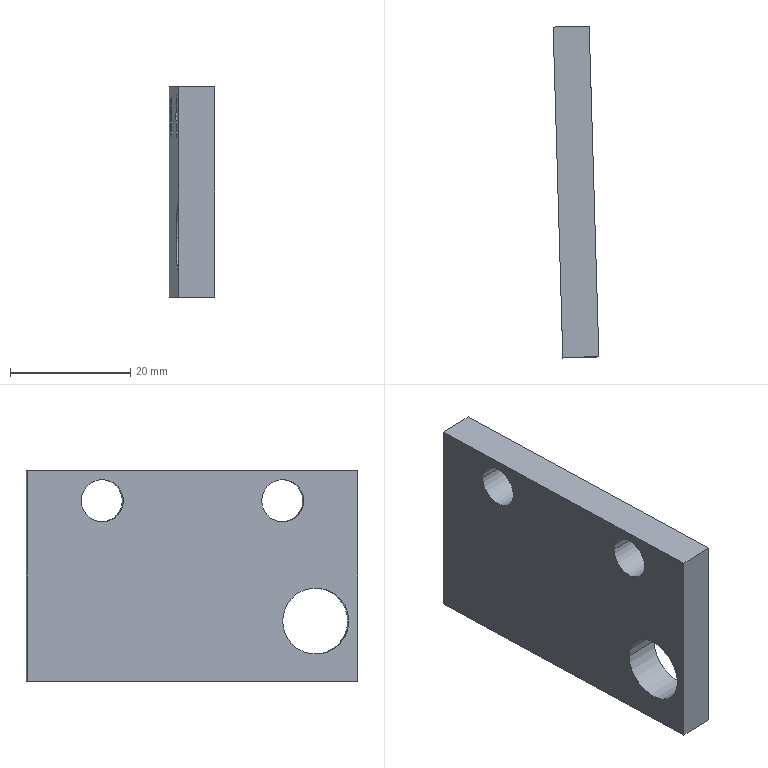Component | SolidWorks | BufferPad-2 | 1 solid | 12 faces | box 7.6 x 55.15 x 35 mm | volume 10518 mm3 | cylinder 6 | plane 6 | commonest cylinder face diameters 7 x4 11 x2 | material 6063
build123d program:
from build123d import *

# Parameters (mm, degrees)
SKETCH1_W           = 55
SKETCH1_H           = 35
BOSS_EXTRUDE1_DEPTH = 6
SKETCH2_R           = 3.5
CUT_EXTRUDE1_DEPTH  = 34.144
SKETCH3_R           = 5.5
CUT_EXTRUDE2_DEPTH  = 34.144


with BuildPart() as part:
    # Sketch1 → Boss-Extrude1 (new body)
    with BuildSketch(Plane.XY):
        Rectangle(SKETCH1_W, SKETCH1_H)
    extrude(amount=BOSS_EXTRUDE1_DEPTH)

    # Sketch2 → Cut-Extrude1 (cut, through all)
    with BuildSketch(Plane.XY.offset(6)):
        with Locations((-15, -12.5)):
            Circle(SKETCH2_R)
        with Locations((15, -12.5)):
            Circle(SKETCH2_R)
    extrude(amount=-CUT_EXTRUDE1_DEPTH, mode=Mode.SUBTRACT)

    # Sketch3 → Cut-Extrude2 (cut, through all)
    with BuildSketch(Plane.XY.offset(6)):
        with Locations((-20.5, 7.5)):
            Circle(SKETCH3_R)
    extrude(amount=-CUT_EXTRUDE2_DEPTH, mode=Mode.SUBTRACT)


solid = part.part

# Placed as in the assembly
solid = solid.moved(Location((-13.559, -152.418, -1233.71), (90, -88.328, 180)))
STEP:
#1=CARTESIAN_POINT('',(-0.504,-7.024,-48.867));
#2=VERTEX_POINT('',#1);
#3=CARTESIAN_POINT('',(-0.5166,-6.591,-48.867));
#4=VERTEX_POINT('',#3);
#5=CARTESIAN_POINT('',(-0.5103,-6.807,-48.867));
#6=DIRECTION('',(-0.9996,-0.02918,0.));
#7=DIRECTION('',(-0.02918,0.9996,0.));
#8=AXIS2_PLACEMENT_3D('',#5,#6,#7);
#9=CIRCLE('',#8,0.2165);
#10=EDGE_CURVE('',#2,#4,#9,.T.);
#11=ORIENTED_EDGE('',*,*,#10,.F.);
#12=CARTESIAN_POINT('',(-0.7401,-7.031,-48.867));
#13=VERTEX_POINT('',#12);
#14=CARTESIAN_POINT('',(-0.504,-7.024,-48.867));
#15=DIRECTION('',(-0.9996,-0.02918,0.));
#16=VECTOR('',#15,39.37);
#17=LINE('',#14,#16);
#18=EDGE_CURVE('',#2,#13,#17,.T.);
#19=ORIENTED_EDGE('',*,*,#18,.T.);
#20=CARTESIAN_POINT('',(-0.7527,-6.598,-48.867));
#21=VERTEX_POINT('',#20);
#22=CARTESIAN_POINT('',(-0.7464,-6.814,-48.867));
#23=DIRECTION('',(-0.9996,-0.02918,0.));
#24=DIRECTION('',(-0.02918,0.9996,0.));
#25=AXIS2_PLACEMENT_3D('',#22,#23,#24);
#26=CIRCLE('',#25,0.2165);
#27=EDGE_CURVE('',#13,#21,#26,.T.);
#28=ORIENTED_EDGE('',*,*,#27,.T.);
#29=CARTESIAN_POINT('',(-0.5166,-6.591,-48.867));
#30=DIRECTION('',(-0.9996,-0.02918,0.));
#31=VECTOR('',#30,39.37);
#32=LINE('',#29,#31);
#33=EDGE_CURVE('',#4,#21,#32,.T.);
#34=ORIENTED_EDGE('',*,*,#33,.F.);
#35=EDGE_LOOP('',(#11,#19,#28,#34));
#36=FACE_OUTER_BOUND('',#35,.T.);
#37=CARTESIAN_POINT('',(-0.5103,-6.807,-48.867));
#38=DIRECTION('',(-0.9996,-0.02918,0.));
#39=DIRECTION('',(-0.02918,0.9996,0.));
#40=AXIS2_PLACEMENT_3D('',#37,#38,#39);
#41=CYLINDRICAL_SURFACE('',#40,0.2165);
#42=ADVANCED_FACE('',(#36),#41,.F.);
#43=CARTESIAN_POINT('',(-0.547,-5.548,-48.079));
#44=VERTEX_POINT('',#43);
#45=CARTESIAN_POINT('',(-0.5551,-5.273,-48.079));
#46=VERTEX_POINT('',#45);
#47=CARTESIAN_POINT('',(-0.5511,-5.41,-48.079));
#48=DIRECTION('',(-0.9996,-0.02918,0.));
#49=DIRECTION('',(-0.02918,0.9996,0.));
#50=AXIS2_PLACEMENT_3D('',#47,#48,#49);
#51=CIRCLE('',#50,0.1378);
#52=EDGE_CURVE('',#44,#46,#51,.T.);
#53=ORIENTED_EDGE('',*,*,#52,.F.);
#54=CARTESIAN_POINT('',(-0.7832,-5.555,-48.079));
#55=VERTEX_POINT('',#54);
#56=CARTESIAN_POINT('',(-0.547,-5.548,-48.079));
#57=DIRECTION('',(-0.9996,-0.02918,0.));
#58=VECTOR('',#57,39.37);
#59=LINE('',#56,#58);
#60=EDGE_CURVE('',#44,#55,#59,.T.);
#61=ORIENTED_EDGE('',*,*,#60,.T.);
#62=CARTESIAN_POINT('',(-0.7912,-5.28,-48.079));
#63=VERTEX_POINT('',#62);
#64=CARTESIAN_POINT('',(-0.7872,-5.417,-48.079));
#65=DIRECTION('',(-0.9996,-0.02918,0.));
#66=DIRECTION('',(-0.02918,0.9996,0.));
#67=AXIS2_PLACEMENT_3D('',#64,#65,#66);
#68=CIRCLE('',#67,0.1378);
#69=EDGE_CURVE('',#55,#63,#68,.T.);
#70=ORIENTED_EDGE('',*,*,#69,.T.);
#71=CARTESIAN_POINT('',(-0.5551,-5.273,-48.079));
#72=DIRECTION('',(-0.9996,-0.02918,0.));
#73=VECTOR('',#72,39.37);
#74=LINE('',#71,#73);
#75=EDGE_CURVE('',#46,#63,#74,.T.);
#76=ORIENTED_EDGE('',*,*,#75,.F.);
#77=EDGE_LOOP('',(#53,#61,#70,#76));
#78=FACE_OUTER_BOUND('',#77,.T.);
#79=CARTESIAN_POINT('',(-0.5511,-5.41,-48.079));
#80=DIRECTION('',(-0.9996,-0.02918,0.));
#81=DIRECTION('',(-0.02918,0.9996,0.));
#82=AXIS2_PLACEMENT_3D('',#79,#80,#81);
#83=CYLINDRICAL_SURFACE('',#82,0.1378);
#84=ADVANCED_FACE('',(#78),#83,.F.);
#85=CARTESIAN_POINT('',(-0.5126,-6.729,-48.079));
#86=VERTEX_POINT('',#85);
#87=CARTESIAN_POINT('',(-0.5206,-6.453,-48.079));
#88=VERTEX_POINT('',#87);
#89=CARTESIAN_POINT('',(-0.5166,-6.591,-48.079));
#90=DIRECTION('',(-0.9996,-0.02918,0.));
#91=DIRECTION('',(-0.02918,0.9996,0.));
#92=AXIS2_PLACEMENT_3D('',#89,#90,#91);
#93=CIRCLE('',#92,0.1378);
#94=EDGE_CURVE('',#86,#88,#93,.T.);
#95=ORIENTED_EDGE('',*,*,#94,.F.);
#96=CARTESIAN_POINT('',(-0.7487,-6.736,-48.079));
#97=VERTEX_POINT('',#96);
#98=CARTESIAN_POINT('',(-0.5126,-6.729,-48.079));
#99=DIRECTION('',(-0.9996,-0.02918,0.));
#100=VECTOR('',#99,39.37);
#101=LINE('',#98,#100);
#102=EDGE_CURVE('',#86,#97,#101,.T.);
#103=ORIENTED_EDGE('',*,*,#102,.T.);
#104=CARTESIAN_POINT('',(-0.7567,-6.46,-48.079));
#105=VERTEX_POINT('',#104);
#106=CARTESIAN_POINT('',(-0.7527,-6.598,-48.079));
#107=DIRECTION('',(-0.9996,-0.02918,0.));
#108=DIRECTION('',(-0.02918,0.9996,0.));
#109=AXIS2_PLACEMENT_3D('',#106,#107,#108);
#110=CIRCLE('',#109,0.1378);
#111=EDGE_CURVE('',#97,#105,#110,.T.);
#112=ORIENTED_EDGE('',*,*,#111,.T.);
#113=CARTESIAN_POINT('',(-0.5206,-6.453,-48.079));
#114=DIRECTION('',(-0.9996,-0.02918,0.));
#115=VECTOR('',#114,39.37);
#116=LINE('',#113,#115);
#117=EDGE_CURVE('',#88,#105,#116,.T.);
#118=ORIENTED_EDGE('',*,*,#117,.F.);
#119=EDGE_LOOP('',(#95,#103,#112,#118));
#120=FACE_OUTER_BOUND('',#119,.T.);
#121=CARTESIAN_POINT('',(-0.5166,-6.591,-48.079));
#122=DIRECTION('',(-0.9996,-0.02918,0.));
#123=DIRECTION('',(-0.02918,0.9996,0.));
#124=AXIS2_PLACEMENT_3D('',#121,#122,#123);
#125=CYLINDRICAL_SURFACE('',#124,0.1378);
#126=ADVANCED_FACE('',(#120),#125,.F.);
#127=CARTESIAN_POINT('',(-0.5654,-4.919,-47.882));
#128=VERTEX_POINT('',#127);
#129=CARTESIAN_POINT('',(-0.5654,-4.919,-49.26));
#130=VERTEX_POINT('',#129);
#131=CARTESIAN_POINT('',(-0.5654,-4.919,-49.26));
#132=DIRECTION('',(-0.,0.,-1.));
#133=VECTOR('',#132,39.37);
#134=LINE('',#131,#133);
#135=EDGE_CURVE('',#128,#130,#134,.T.);
#136=ORIENTED_EDGE('',*,*,#135,.T.);
#137=CARTESIAN_POINT('',(-0.8015,-4.925,-49.26));
#138=VERTEX_POINT('',#137);
#139=CARTESIAN_POINT('',(-0.8015,-4.925,-49.26));
#140=DIRECTION('',(0.9996,0.02918,-0.));
#141=VECTOR('',#140,39.37);
#142=LINE('',#139,#141);
#143=EDGE_CURVE('',#138,#130,#142,.T.);
#144=ORIENTED_EDGE('',*,*,#143,.F.);
#145=CARTESIAN_POINT('',(-0.8015,-4.925,-47.882));
#146=VERTEX_POINT('',#145);
#147=CARTESIAN_POINT('',(-0.8015,-4.925,-49.26));
#148=DIRECTION('',(-0.,0.,-1.));
#149=VECTOR('',#148,39.37);
#150=LINE('',#147,#149);
#151=EDGE_CURVE('',#146,#138,#150,.T.);
#152=ORIENTED_EDGE('',*,*,#151,.F.);
#153=CARTESIAN_POINT('',(-0.8015,-4.925,-47.882));
#154=DIRECTION('',(0.9996,0.02918,-0.));
#155=VECTOR('',#154,39.37);
#156=LINE('',#153,#155);
#157=EDGE_CURVE('',#146,#128,#156,.T.);
#158=ORIENTED_EDGE('',*,*,#157,.T.);
#159=EDGE_LOOP('',(#136,#144,#152,#158));
#160=FACE_OUTER_BOUND('',#159,.T.);
#161=CARTESIAN_POINT('',(-0.8015,-4.925,-49.26));
#162=DIRECTION('',(0.02918,-0.9996,-0.));
#163=DIRECTION('',(0.,-0.,1.));
#164=AXIS2_PLACEMENT_3D('',#161,#162,#163);
#165=PLANE('',#164);
#166=ADVANCED_FACE('',(#160),#165,.F.);
#167=CARTESIAN_POINT('',(-0.5022,-7.083,-49.26));
#168=VERTEX_POINT('',#167);
#169=CARTESIAN_POINT('',(-0.5022,-7.083,-49.26));
#170=DIRECTION('',(0.02918,-0.9996,-0.));
#171=VECTOR('',#170,39.37);
#172=LINE('',#169,#171);
#173=EDGE_CURVE('',#130,#168,#172,.T.);
#174=ORIENTED_EDGE('',*,*,#173,.T.);
#175=CARTESIAN_POINT('',(-0.7384,-7.09,-49.26));
#176=VERTEX_POINT('',#175);
#177=CARTESIAN_POINT('',(-0.7384,-7.09,-49.26));
#178=DIRECTION('',(0.9996,0.02918,-0.));
#179=VECTOR('',#178,39.37);
#180=LINE('',#177,#179);
#181=EDGE_CURVE('',#176,#168,#180,.T.);
#182=ORIENTED_EDGE('',*,*,#181,.F.);
#183=CARTESIAN_POINT('',(-0.7384,-7.09,-49.26));
#184=DIRECTION('',(0.02918,-0.9996,-0.));
#185=VECTOR('',#184,39.37);
#186=LINE('',#183,#185);
#187=EDGE_CURVE('',#138,#176,#186,.T.);
#188=ORIENTED_EDGE('',*,*,#187,.F.);
#189=ORIENTED_EDGE('',*,*,#143,.T.);
#190=EDGE_LOOP('',(#174,#182,#188,#189));
#191=FACE_OUTER_BOUND('',#190,.T.);
#192=CARTESIAN_POINT('',(-0.7384,-7.09,-49.26));
#193=DIRECTION('',(0.,-0.,1.));
#194=DIRECTION('',(0.9996,0.02918,-0.));
#195=AXIS2_PLACEMENT_3D('',#192,#193,#194);
#196=PLANE('',#195);
#197=ADVANCED_FACE('',(#191),#196,.F.);
#198=CARTESIAN_POINT('',(-0.5022,-7.083,-47.882));
#199=VERTEX_POINT('',#198);
#200=CARTESIAN_POINT('',(-0.5022,-7.083,-49.26));
#201=DIRECTION('',(0.,-0.,1.));
#202=VECTOR('',#201,39.37);
#203=LINE('',#200,#202);
#204=EDGE_CURVE('',#168,#199,#203,.T.);
#205=ORIENTED_EDGE('',*,*,#204,.T.);
#206=CARTESIAN_POINT('',(-0.7384,-7.09,-47.882));
#207=VERTEX_POINT('',#206);
#208=CARTESIAN_POINT('',(-0.7384,-7.09,-47.882));
#209=DIRECTION('',(0.9996,0.02918,-0.));
#210=VECTOR('',#209,39.37);
#211=LINE('',#208,#210);
#212=EDGE_CURVE('',#207,#199,#211,.T.);
#213=ORIENTED_EDGE('',*,*,#212,.F.);
#214=CARTESIAN_POINT('',(-0.7384,-7.09,-49.26));
#215=DIRECTION('',(0.,-0.,1.));
#216=VECTOR('',#215,39.37);
#217=LINE('',#214,#216);
#218=EDGE_CURVE('',#176,#207,#217,.T.);
#219=ORIENTED_EDGE('',*,*,#218,.F.);
#220=ORIENTED_EDGE('',*,*,#181,.T.);
#221=EDGE_LOOP('',(#205,#213,#219,#220));
#222=FACE_OUTER_BOUND('',#221,.T.);
#223=CARTESIAN_POINT('',(-0.7384,-7.09,-49.26));
#224=DIRECTION('',(-0.02918,0.9996,0.));
#225=DIRECTION('',(-0.,0.,-1.));
#226=AXIS2_PLACEMENT_3D('',#223,#224,#225);
#227=PLANE('',#226);
#228=ADVANCED_FACE('',(#222),#227,.F.);
#229=CARTESIAN_POINT('',(-0.5022,-7.083,-47.882));
#230=DIRECTION('',(-0.02918,0.9996,0.));
#231=VECTOR('',#230,39.37);
#232=LINE('',#229,#231);
#233=EDGE_CURVE('',#199,#128,#232,.T.);
#234=ORIENTED_EDGE('',*,*,#233,.T.);
#235=ORIENTED_EDGE('',*,*,#157,.F.);
#236=CARTESIAN_POINT('',(-0.7384,-7.09,-47.882));
#237=DIRECTION('',(-0.02918,0.9996,0.));
#238=VECTOR('',#237,39.37);
#239=LINE('',#236,#238);
#240=EDGE_CURVE('',#207,#146,#239,.T.);
#241=ORIENTED_EDGE('',*,*,#240,.F.);
#242=ORIENTED_EDGE('',*,*,#212,.T.);
#243=EDGE_LOOP('',(#234,#235,#241,#242));
#244=FACE_OUTER_BOUND('',#243,.T.);
#245=CARTESIAN_POINT('',(-0.7384,-7.09,-47.882));
#246=DIRECTION('',(-0.,0.,-1.));
#247=DIRECTION('',(-0.9996,-0.02918,0.));
#248=AXIS2_PLACEMENT_3D('',#245,#246,#247);
#249=PLANE('',#248);
#250=ADVANCED_FACE('',(#244),#249,.F.);
#251=CARTESIAN_POINT('',(-0.7464,-6.814,-48.867));
#252=DIRECTION('',(-0.9996,-0.02918,0.));
#253=DIRECTION('',(-0.02918,0.9996,0.));
#254=AXIS2_PLACEMENT_3D('',#251,#252,#253);
#255=CIRCLE('',#254,0.2165);
#256=EDGE_CURVE('',#21,#13,#255,.T.);
#257=ORIENTED_EDGE('',*,*,#256,.F.);
#258=ORIENTED_EDGE('',*,*,#27,.F.);
#259=EDGE_LOOP('',(#257,#258));
#260=FACE_BOUND('',#259,.T.);
#261=CARTESIAN_POINT('',(-0.7872,-5.417,-48.079));
#262=DIRECTION('',(-0.9996,-0.02918,0.));
#263=DIRECTION('',(-0.02918,0.9996,0.));
#264=AXIS2_PLACEMENT_3D('',#261,#262,#263);
#265=CIRCLE('',#264,0.1378);
#266=EDGE_CURVE('',#63,#55,#265,.T.);
#267=ORIENTED_EDGE('',*,*,#266,.F.);
#268=ORIENTED_EDGE('',*,*,#69,.F.);
#269=EDGE_LOOP('',(#267,#268));
#270=FACE_BOUND('',#269,.T.);
#271=CARTESIAN_POINT('',(-0.7527,-6.598,-48.079));
#272=DIRECTION('',(-0.9996,-0.02918,0.));
#273=DIRECTION('',(-0.02918,0.9996,0.));
#274=AXIS2_PLACEMENT_3D('',#271,#272,#273);
#275=CIRCLE('',#274,0.1378);
#276=EDGE_CURVE('',#105,#97,#275,.T.);
#277=ORIENTED_EDGE('',*,*,#276,.F.);
#278=ORIENTED_EDGE('',*,*,#111,.F.);
#279=EDGE_LOOP('',(#277,#278));
#280=FACE_BOUND('',#279,.T.);
#281=ORIENTED_EDGE('',*,*,#151,.T.);
#282=ORIENTED_EDGE('',*,*,#187,.T.);
#283=ORIENTED_EDGE('',*,*,#218,.T.);
#284=ORIENTED_EDGE('',*,*,#240,.T.);
#285=EDGE_LOOP('',(#281,#282,#283,#284));
#286=FACE_OUTER_BOUND('',#285,.T.);
#287=CARTESIAN_POINT('',(-0.77,-6.008,-48.571));
#288=DIRECTION('',(-0.9996,-0.02918,0.));
#289=DIRECTION('',(-0.02918,0.9996,0.));
#290=AXIS2_PLACEMENT_3D('',#287,#288,#289);
#291=PLANE('',#290);
#292=ADVANCED_FACE('',(#260,#270,#280,#286),#291,.T.);
#293=CARTESIAN_POINT('',(-0.5103,-6.807,-48.867));
#294=DIRECTION('',(-0.9996,-0.02918,0.));
#295=DIRECTION('',(-0.02918,0.9996,0.));
#296=AXIS2_PLACEMENT_3D('',#293,#294,#295);
#297=CIRCLE('',#296,0.2165);
#298=EDGE_CURVE('',#4,#2,#297,.T.);
#299=ORIENTED_EDGE('',*,*,#298,.T.);
#300=ORIENTED_EDGE('',*,*,#10,.T.);
#301=EDGE_LOOP('',(#299,#300));
#302=FACE_BOUND('',#301,.T.);
#303=CARTESIAN_POINT('',(-0.5511,-5.41,-48.079));
#304=DIRECTION('',(-0.9996,-0.02918,0.));
#305=DIRECTION('',(-0.02918,0.9996,0.));
#306=AXIS2_PLACEMENT_3D('',#303,#304,#305);
#307=CIRCLE('',#306,0.1378);
#308=EDGE_CURVE('',#46,#44,#307,.T.);
#309=ORIENTED_EDGE('',*,*,#308,.T.);
#310=ORIENTED_EDGE('',*,*,#52,.T.);
#311=EDGE_LOOP('',(#309,#310));
#312=FACE_BOUND('',#311,.T.);
#313=CARTESIAN_POINT('',(-0.5166,-6.591,-48.079));
#314=DIRECTION('',(-0.9996,-0.02918,0.));
#315=DIRECTION('',(-0.02918,0.9996,0.));
#316=AXIS2_PLACEMENT_3D('',#313,#314,#315);
#317=CIRCLE('',#316,0.1378);
#318=EDGE_CURVE('',#88,#86,#317,.T.);
#319=ORIENTED_EDGE('',*,*,#318,.T.);
#320=ORIENTED_EDGE('',*,*,#94,.T.);
#321=EDGE_LOOP('',(#319,#320));
#322=FACE_BOUND('',#321,.T.);
#323=ORIENTED_EDGE('',*,*,#135,.F.);
#324=ORIENTED_EDGE('',*,*,#233,.F.);
#325=ORIENTED_EDGE('',*,*,#204,.F.);
#326=ORIENTED_EDGE('',*,*,#173,.F.);
#327=EDGE_LOOP('',(#323,#324,#325,#326));
#328=FACE_OUTER_BOUND('',#327,.T.);
#329=CARTESIAN_POINT('',(-0.5338,-6.001,-48.571));
#330=DIRECTION('',(-0.9996,-0.02918,0.));
#331=DIRECTION('',(-0.02918,0.9996,0.));
#332=AXIS2_PLACEMENT_3D('',#329,#330,#331);
#333=PLANE('',#332);
#334=ADVANCED_FACE('',(#302,#312,#322,#328),#333,.F.);
#335=ORIENTED_EDGE('',*,*,#102,.F.);
#336=ORIENTED_EDGE('',*,*,#318,.F.);
#337=ORIENTED_EDGE('',*,*,#117,.T.);
#338=ORIENTED_EDGE('',*,*,#276,.T.);
#339=EDGE_LOOP('',(#335,#336,#337,#338));
#340=FACE_OUTER_BOUND('',#339,.T.);
#341=CARTESIAN_POINT('',(-0.5166,-6.591,-48.079));
#342=DIRECTION('',(-0.9996,-0.02918,0.));
#343=DIRECTION('',(-0.02918,0.9996,0.));
#344=AXIS2_PLACEMENT_3D('',#341,#342,#343);
#345=CYLINDRICAL_SURFACE('',#344,0.1378);
#346=ADVANCED_FACE('',(#340),#345,.F.);
#347=ORIENTED_EDGE('',*,*,#60,.F.);
#348=ORIENTED_EDGE('',*,*,#308,.F.);
#349=ORIENTED_EDGE('',*,*,#75,.T.);
#350=ORIENTED_EDGE('',*,*,#266,.T.);
#351=EDGE_LOOP('',(#347,#348,#349,#350));
#352=FACE_OUTER_BOUND('',#351,.T.);
#353=CARTESIAN_POINT('',(-0.5511,-5.41,-48.079));
#354=DIRECTION('',(-0.9996,-0.02918,0.));
#355=DIRECTION('',(-0.02918,0.9996,0.));
#356=AXIS2_PLACEMENT_3D('',#353,#354,#355);
#357=CYLINDRICAL_SURFACE('',#356,0.1378);
#358=ADVANCED_FACE('',(#352),#357,.F.);
#359=ORIENTED_EDGE('',*,*,#18,.F.);
#360=ORIENTED_EDGE('',*,*,#298,.F.);
#361=ORIENTED_EDGE('',*,*,#33,.T.);
#362=ORIENTED_EDGE('',*,*,#256,.T.);
#363=EDGE_LOOP('',(#359,#360,#361,#362));
#364=FACE_OUTER_BOUND('',#363,.T.);
#365=CARTESIAN_POINT('',(-0.5103,-6.807,-48.867));
#366=DIRECTION('',(-0.9996,-0.02918,0.));
#367=DIRECTION('',(-0.02918,0.9996,0.));
#368=AXIS2_PLACEMENT_3D('',#365,#366,#367);
#369=CYLINDRICAL_SURFACE('',#368,0.2165);
#370=ADVANCED_FACE('',(#364),#369,.F.);
#371=CLOSED_SHELL('',(#42,#84,#126,#166,#197,#228,#250,#292,#334,#346,#358,#370));
#372=MANIFOLD_SOLID_BREP('',#371);
#373=CARTESIAN_POINT('',(0.,0.,0.));
#374=DIRECTION('',(0.,0.,1.));
#375=DIRECTION('',(1.,0.,0.));
#376=AXIS2_PLACEMENT_3D('',#373,#374,#375);
#377=(LENGTH_UNIT()NAMED_UNIT(*)SI_UNIT($,.METRE.));
#378=LENGTH_MEASURE_WITH_UNIT(LENGTH_MEASURE(0.0254),#377);
#379=DIMENSIONAL_EXPONENTS(1.,0.,0.,0.,0.,0.,0.);
#380=(CONVERSION_BASED_UNIT('',#378)LENGTH_UNIT()NAMED_UNIT(#379));
#381=UNCERTAINTY_MEASURE_WITH_UNIT(LENGTH_MEASURE(0.00001),#380,'','');
#382=(NAMED_UNIT(*)PLANE_ANGLE_UNIT()SI_UNIT($,.RADIAN.));
#383=(NAMED_UNIT(*)SI_UNIT($,.STERADIAN.)SOLID_ANGLE_UNIT());
#384=(GEOMETRIC_REPRESENTATION_CONTEXT(3)GLOBAL_UNCERTAINTY_ASSIGNED_CONTEXT((#381))GLOBAL_UNIT_ASSIGNED_CONTEXT((#380,#382,#383))REPRESENTATION_CONTEXT('',''));
#385=ADVANCED_BREP_SHAPE_REPRESENTATION('',(#372,#376),#384);
#386=COLOUR_RGB('',0.7922,0.8196,0.9333);
#387=FILL_AREA_STYLE_COLOUR('',#386);
#388=FILL_AREA_STYLE('',(#387));
#389=SURFACE_STYLE_FILL_AREA(#388);
#390=SURFACE_SIDE_STYLE('',(#389));
#391=SURFACE_STYLE_USAGE(.BOTH.,#390);
#392=PRESENTATION_STYLE_ASSIGNMENT((#391));
#393=STYLED_ITEM('',(#392),#372);
#394=PRESENTATION_LAYER_ASSIGNMENT('','',(#393));
#395=(LENGTH_UNIT()NAMED_UNIT(*)SI_UNIT($,.METRE.));
#396=LENGTH_MEASURE_WITH_UNIT(LENGTH_MEASURE(0.0254),#395);
#397=DIMENSIONAL_EXPONENTS(1.,0.,0.,0.,0.,0.,0.);
#398=(CONVERSION_BASED_UNIT('',#396)LENGTH_UNIT()NAMED_UNIT(#397));
#399=UNCERTAINTY_MEASURE_WITH_UNIT(LENGTH_MEASURE(0.00001),#398,'','');
#400=(NAMED_UNIT(*)PLANE_ANGLE_UNIT()SI_UNIT($,.RADIAN.));
#401=(NAMED_UNIT(*)SI_UNIT($,.STERADIAN.)SOLID_ANGLE_UNIT());
#402=(GEOMETRIC_REPRESENTATION_CONTEXT(3)GLOBAL_UNCERTAINTY_ASSIGNED_CONTEXT((#399))GLOBAL_UNIT_ASSIGNED_CONTEXT((#398,#400,#401))REPRESENTATION_CONTEXT('',''));
#403=MECHANICAL_DESIGN_GEOMETRIC_PRESENTATION_REPRESENTATION('',(#393),#402);